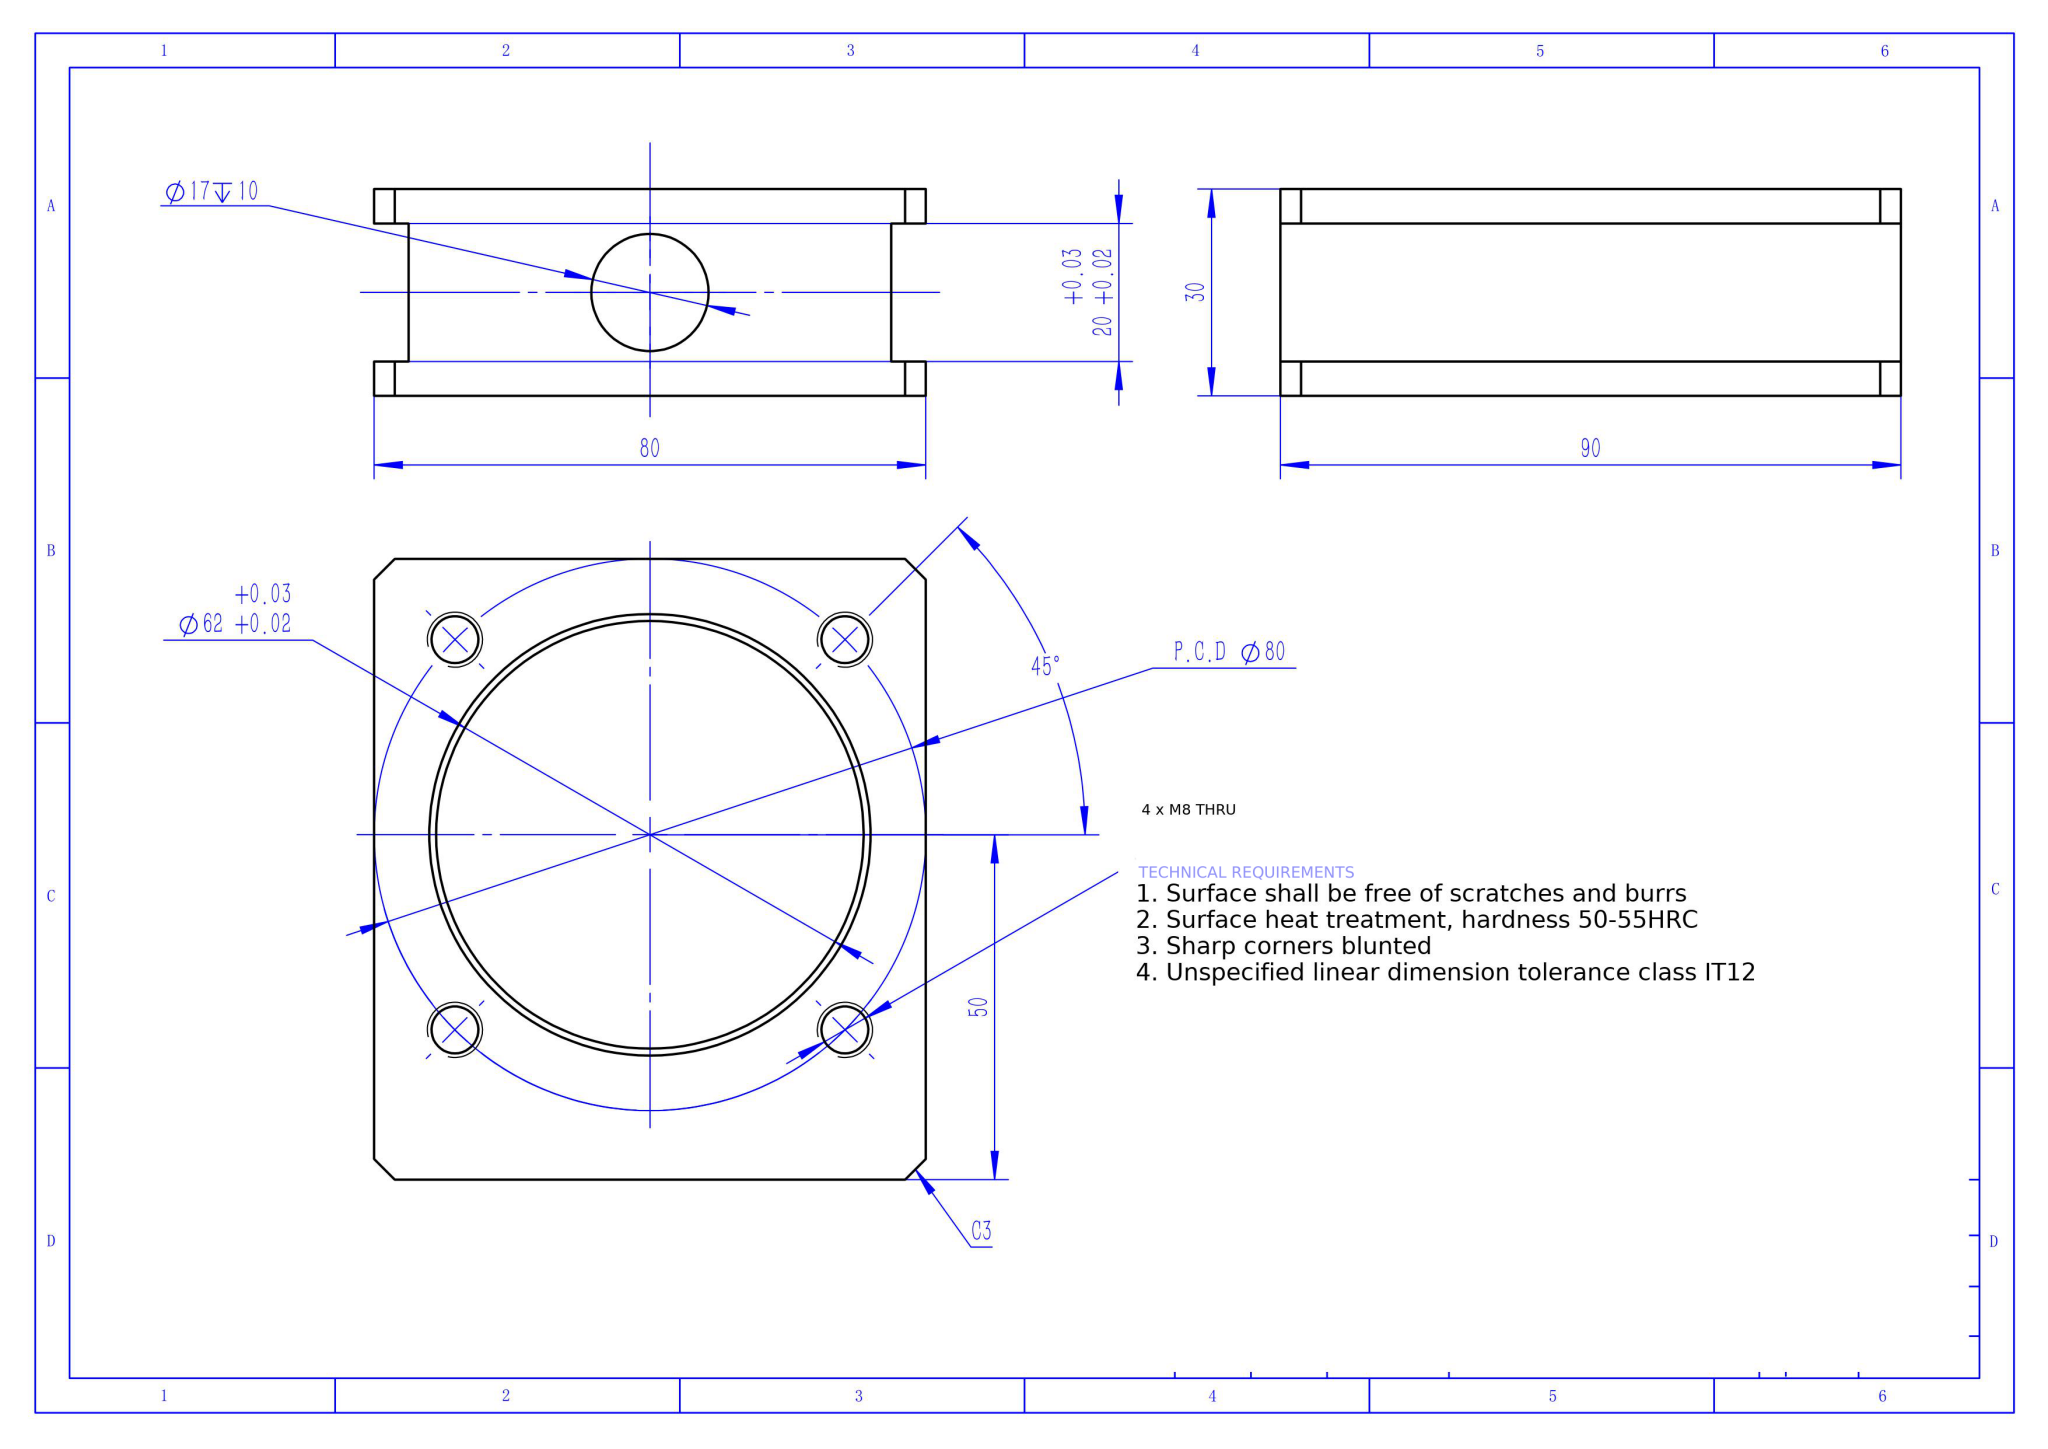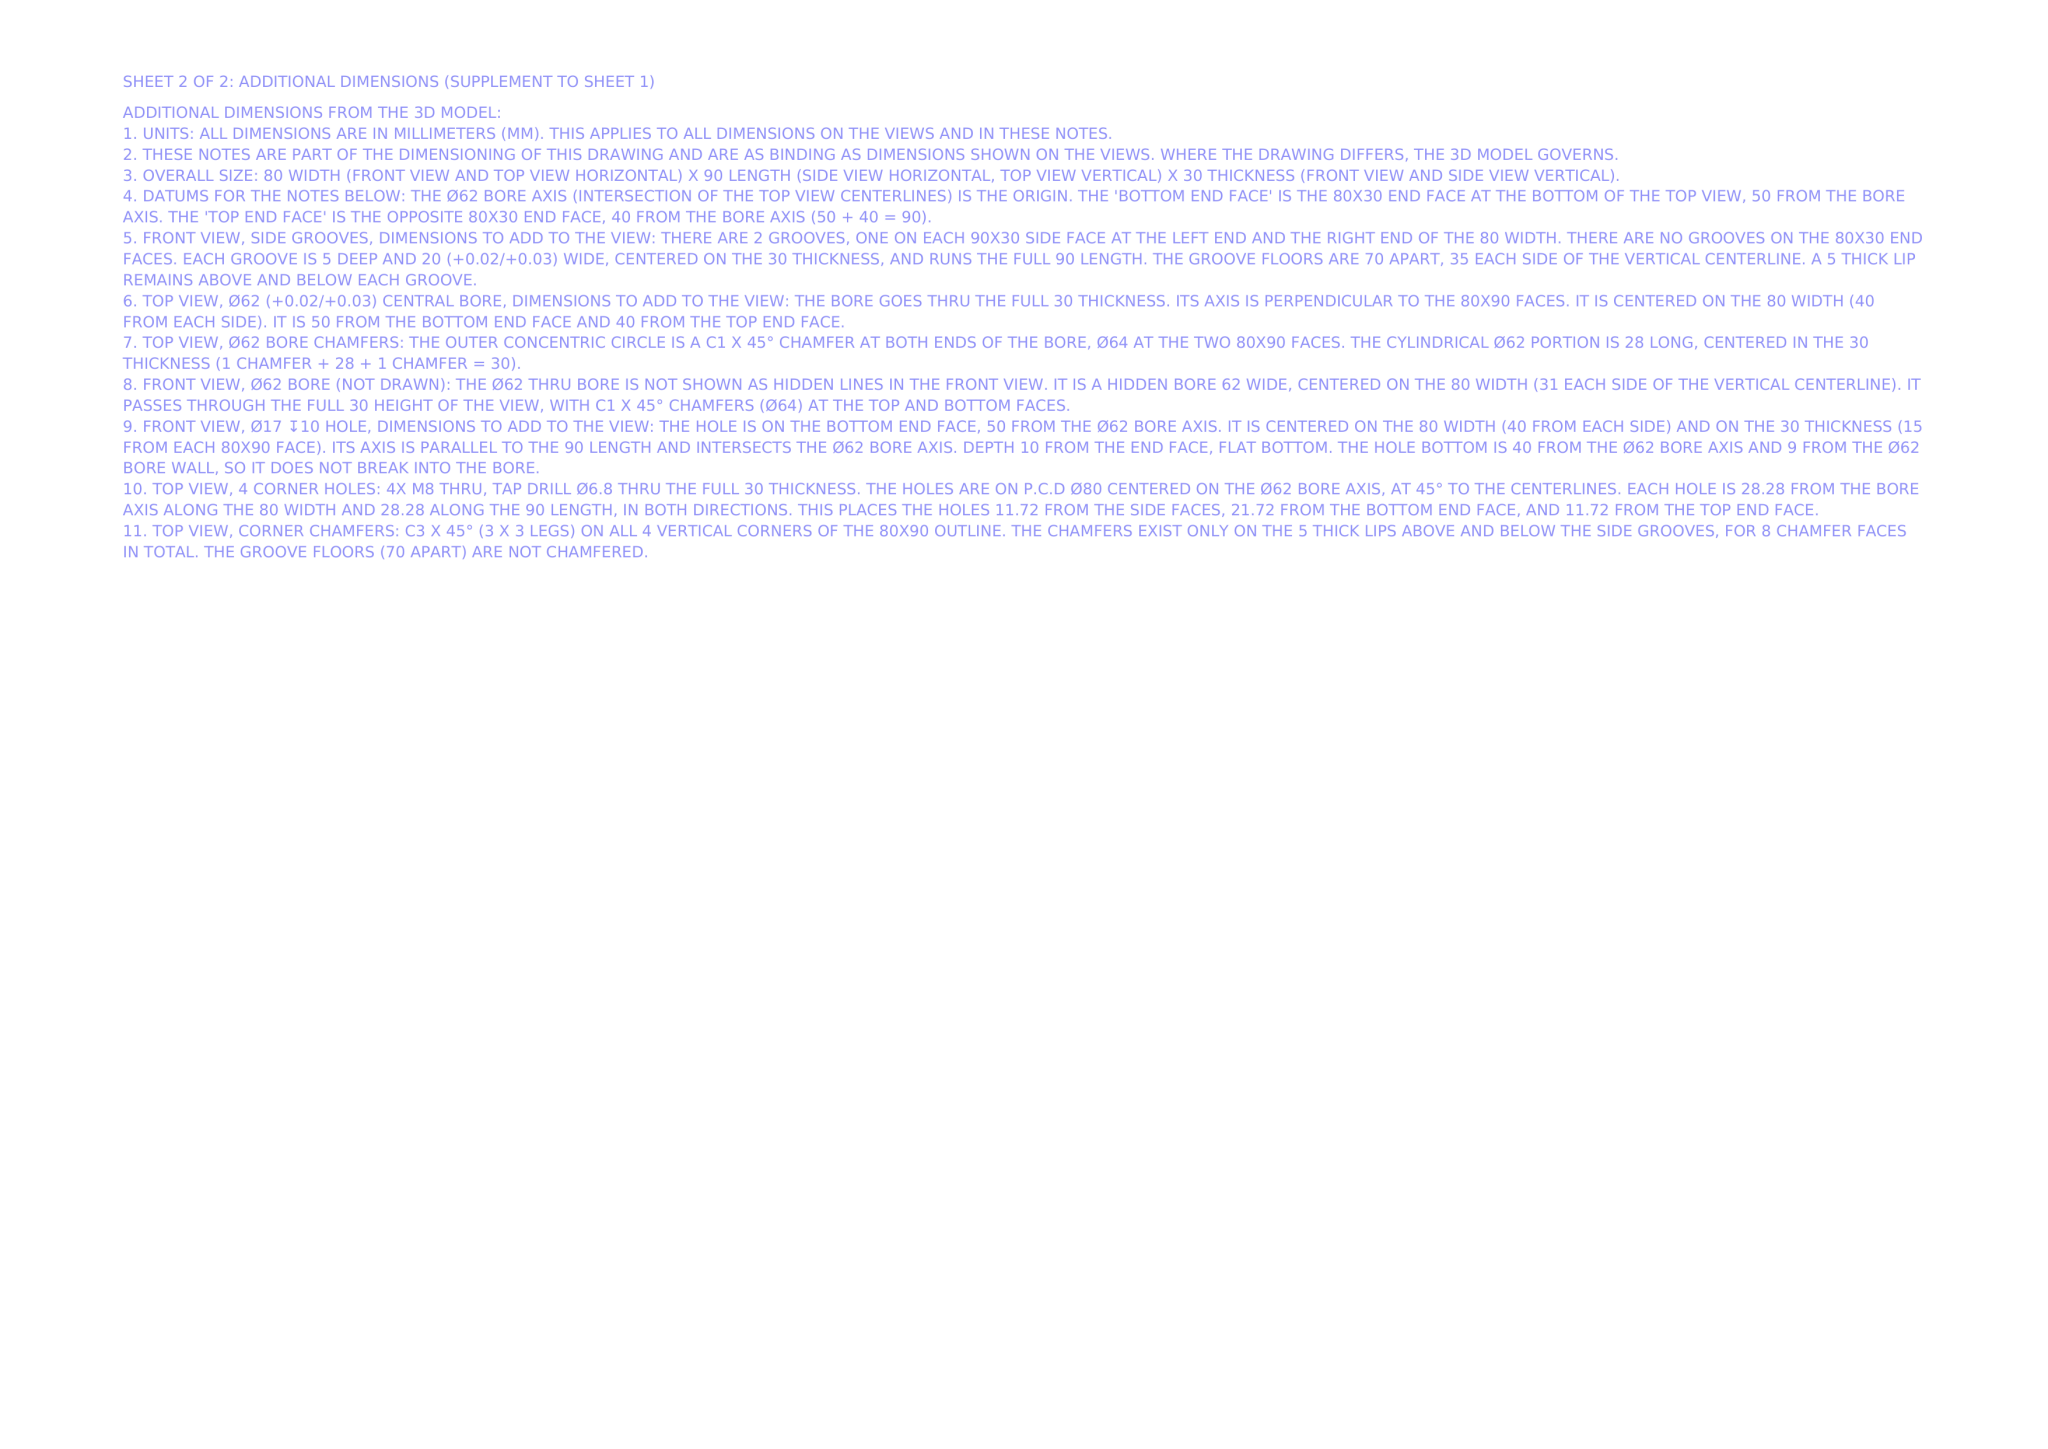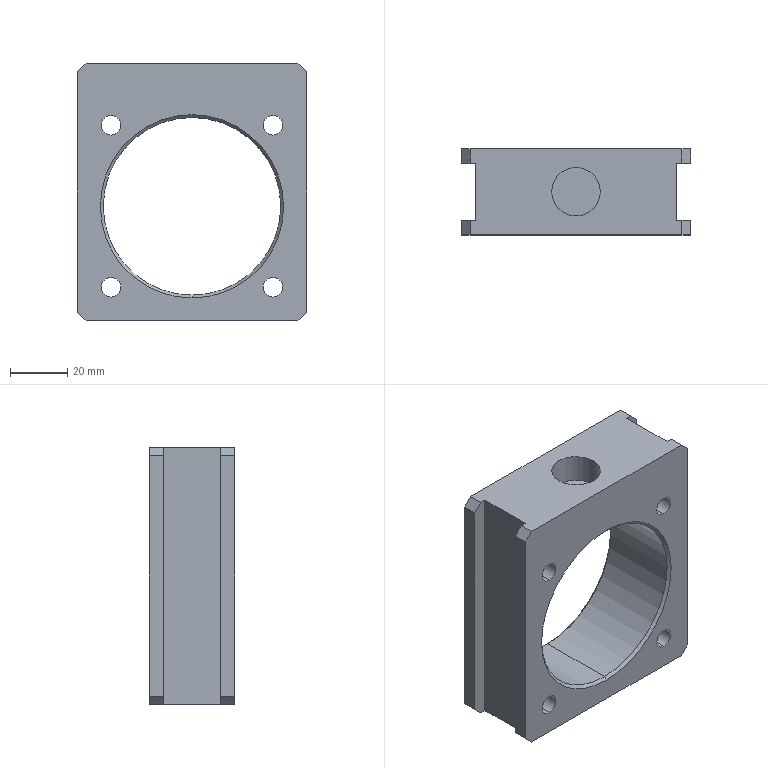Part | NX | mm | 1 solid | 39 faces | box 80 x 30 x 90 mm | volume 100423 mm3 | plane 23 | cylinder 12 | cone 4 | commonest cylinder face diameters 6.8 x8 17 x2 62 x2